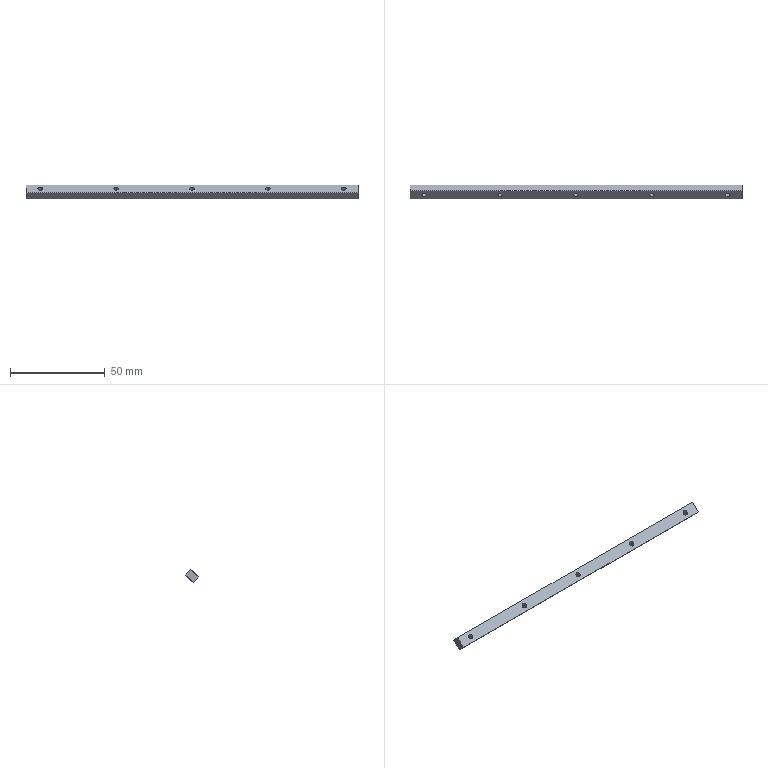Component | SolidWorks | FlatKey6-175-1 | 1 solid | 16 faces | box 175 x 7.31 x 7.25 mm | volume 4409 mm3 | cylinder 10 | plane 6 | commonest cylinder face diameters 2.5 x10 | material Alternative Material
build123d program:
from build123d import *

# Parameters (mm, degrees)
SKETCH1_W           = 175
SKETCH1_H           = 6
BOSS_EXTRUDE1_DEPTH = 4.3
M3_TAPPED_HOLE1_D   = 2.5


with BuildPart() as part:
    # Sketch1 → Boss-Extrude1 (new body)
    with BuildSketch(Plane.XY):
        Rectangle(SKETCH1_W, SKETCH1_H)
    extrude(amount=BOSS_EXTRUDE1_DEPTH)

    # M3 Tapped Hole1 (through all)
    with Locations(Plane.XY.offset(4.3)):
        with Locations((-80, 0), (-40, 0), (0, 0), (40, 0), (80, 0)):
            Hole(M3_TAPPED_HOLE1_D / 2)


solid = part.part

# Placed as in the assembly
solid = solid.moved(Location((-53.09, -33.192, -12.39), (43.57, 0, 0)))
STEP:
#1=COLOUR_RGB('',0.7922,0.8196,0.9333);
#2=FILL_AREA_STYLE_COLOUR('',#1);
#3=FILL_AREA_STYLE('',(#2));
#4=SURFACE_STYLE_FILL_AREA(#3);
#5=SURFACE_SIDE_STYLE('',(#4));
#6=SURFACE_STYLE_USAGE(.BOTH.,#5);
#7=PRESENTATION_STYLE_ASSIGNMENT((#6));
#8=CARTESIAN_POINT('',(-5.289,-1.423,-0.3652));
#9=VERTEX_POINT('',#8);
#10=CARTESIAN_POINT('',(-5.191,-1.423,-0.3652));
#11=VERTEX_POINT('',#10);
#12=CARTESIAN_POINT('',(-5.24,-1.423,-0.3652));
#13=DIRECTION('',(0.,0.6892,-0.7245));
#14=DIRECTION('',(1.,0.,0.));
#15=AXIS2_PLACEMENT_3D('',#12,#13,#14);
#16=CIRCLE('',#15,0.04921);
#17=EDGE_CURVE('',#9,#11,#16,.T.);
#18=ORIENTED_EDGE('',*,*,#17,.F.);
#19=CARTESIAN_POINT('',(-5.289,-1.307,-0.4878));
#20=VERTEX_POINT('',#19);
#21=CARTESIAN_POINT('',(-5.289,-1.307,-0.4878));
#22=DIRECTION('',(0.,0.6892,-0.7245));
#23=VECTOR('',#22,39.37);
#24=LINE('',#21,#23);
#25=EDGE_CURVE('',#9,#20,#24,.T.);
#26=ORIENTED_EDGE('',*,*,#25,.T.);
#27=CARTESIAN_POINT('',(-5.191,-1.307,-0.4878));
#28=VERTEX_POINT('',#27);
#29=CARTESIAN_POINT('',(-5.24,-1.307,-0.4878));
#30=DIRECTION('',(0.,0.6892,-0.7245));
#31=DIRECTION('',(1.,0.,0.));
#32=AXIS2_PLACEMENT_3D('',#29,#30,#31);
#33=CIRCLE('',#32,0.04921);
#34=EDGE_CURVE('',#20,#28,#33,.T.);
#35=ORIENTED_EDGE('',*,*,#34,.T.);
#36=CARTESIAN_POINT('',(-5.191,-1.307,-0.4878));
#37=DIRECTION('',(0.,0.6892,-0.7245));
#38=VECTOR('',#37,39.37);
#39=LINE('',#36,#38);
#40=EDGE_CURVE('',#11,#28,#39,.T.);
#41=ORIENTED_EDGE('',*,*,#40,.F.);
#42=EDGE_LOOP('',(#18,#26,#35,#41));
#43=FACE_OUTER_BOUND('',#42,.T.);
#44=CARTESIAN_POINT('',(-5.24,-1.307,-0.4878));
#45=DIRECTION('',(0.,0.6892,-0.7245));
#46=DIRECTION('',(1.,0.,0.));
#47=AXIS2_PLACEMENT_3D('',#44,#45,#46);
#48=CYLINDRICAL_SURFACE('',#47,0.04921);
#49=ADVANCED_FACE('',(#43),#48,.F.);
#50=CARTESIAN_POINT('',(-3.714,-1.423,-0.3652));
#51=VERTEX_POINT('',#50);
#52=CARTESIAN_POINT('',(-3.616,-1.423,-0.3652));
#53=VERTEX_POINT('',#52);
#54=CARTESIAN_POINT('',(-3.665,-1.423,-0.3652));
#55=DIRECTION('',(0.,0.6892,-0.7245));
#56=DIRECTION('',(1.,0.,0.));
#57=AXIS2_PLACEMENT_3D('',#54,#55,#56);
#58=CIRCLE('',#57,0.04921);
#59=EDGE_CURVE('',#51,#53,#58,.T.);
#60=ORIENTED_EDGE('',*,*,#59,.F.);
#61=CARTESIAN_POINT('',(-3.714,-1.307,-0.4878));
#62=VERTEX_POINT('',#61);
#63=CARTESIAN_POINT('',(-3.714,-1.307,-0.4878));
#64=DIRECTION('',(0.,0.6892,-0.7245));
#65=VECTOR('',#64,39.37);
#66=LINE('',#63,#65);
#67=EDGE_CURVE('',#51,#62,#66,.T.);
#68=ORIENTED_EDGE('',*,*,#67,.T.);
#69=CARTESIAN_POINT('',(-3.616,-1.307,-0.4878));
#70=VERTEX_POINT('',#69);
#71=CARTESIAN_POINT('',(-3.665,-1.307,-0.4878));
#72=DIRECTION('',(0.,0.6892,-0.7245));
#73=DIRECTION('',(1.,0.,0.));
#74=AXIS2_PLACEMENT_3D('',#71,#72,#73);
#75=CIRCLE('',#74,0.04921);
#76=EDGE_CURVE('',#62,#70,#75,.T.);
#77=ORIENTED_EDGE('',*,*,#76,.T.);
#78=CARTESIAN_POINT('',(-3.616,-1.307,-0.4878));
#79=DIRECTION('',(0.,0.6892,-0.7245));
#80=VECTOR('',#79,39.37);
#81=LINE('',#78,#80);
#82=EDGE_CURVE('',#53,#70,#81,.T.);
#83=ORIENTED_EDGE('',*,*,#82,.F.);
#84=EDGE_LOOP('',(#60,#68,#77,#83));
#85=FACE_OUTER_BOUND('',#84,.T.);
#86=CARTESIAN_POINT('',(-3.665,-1.307,-0.4878));
#87=DIRECTION('',(0.,0.6892,-0.7245));
#88=DIRECTION('',(1.,0.,0.));
#89=AXIS2_PLACEMENT_3D('',#86,#87,#88);
#90=CYLINDRICAL_SURFACE('',#89,0.04921);
#91=ADVANCED_FACE('',(#85),#90,.F.);
#92=CARTESIAN_POINT('',(-2.139,-1.423,-0.3652));
#93=VERTEX_POINT('',#92);
#94=CARTESIAN_POINT('',(-2.041,-1.423,-0.3652));
#95=VERTEX_POINT('',#94);
#96=CARTESIAN_POINT('',(-2.09,-1.423,-0.3652));
#97=DIRECTION('',(0.,0.6892,-0.7245));
#98=DIRECTION('',(1.,0.,0.));
#99=AXIS2_PLACEMENT_3D('',#96,#97,#98);
#100=CIRCLE('',#99,0.04921);
#101=EDGE_CURVE('',#93,#95,#100,.T.);
#102=ORIENTED_EDGE('',*,*,#101,.F.);
#103=CARTESIAN_POINT('',(-2.139,-1.307,-0.4878));
#104=VERTEX_POINT('',#103);
#105=CARTESIAN_POINT('',(-2.139,-1.307,-0.4878));
#106=DIRECTION('',(0.,0.6892,-0.7245));
#107=VECTOR('',#106,39.37);
#108=LINE('',#105,#107);
#109=EDGE_CURVE('',#93,#104,#108,.T.);
#110=ORIENTED_EDGE('',*,*,#109,.T.);
#111=CARTESIAN_POINT('',(-2.041,-1.307,-0.4878));
#112=VERTEX_POINT('',#111);
#113=CARTESIAN_POINT('',(-2.09,-1.307,-0.4878));
#114=DIRECTION('',(0.,0.6892,-0.7245));
#115=DIRECTION('',(1.,0.,0.));
#116=AXIS2_PLACEMENT_3D('',#113,#114,#115);
#117=CIRCLE('',#116,0.04921);
#118=EDGE_CURVE('',#104,#112,#117,.T.);
#119=ORIENTED_EDGE('',*,*,#118,.T.);
#120=CARTESIAN_POINT('',(-2.041,-1.307,-0.4878));
#121=DIRECTION('',(0.,0.6892,-0.7245));
#122=VECTOR('',#121,39.37);
#123=LINE('',#120,#122);
#124=EDGE_CURVE('',#95,#112,#123,.T.);
#125=ORIENTED_EDGE('',*,*,#124,.F.);
#126=EDGE_LOOP('',(#102,#110,#119,#125));
#127=FACE_OUTER_BOUND('',#126,.T.);
#128=CARTESIAN_POINT('',(-2.09,-1.307,-0.4878));
#129=DIRECTION('',(0.,0.6892,-0.7245));
#130=DIRECTION('',(1.,0.,0.));
#131=AXIS2_PLACEMENT_3D('',#128,#129,#130);
#132=CYLINDRICAL_SURFACE('',#131,0.04921);
#133=ADVANCED_FACE('',(#127),#132,.F.);
#134=CARTESIAN_POINT('',(-0.5646,-1.423,-0.3652));
#135=VERTEX_POINT('',#134);
#136=CARTESIAN_POINT('',(-0.4662,-1.423,-0.3652));
#137=VERTEX_POINT('',#136);
#138=CARTESIAN_POINT('',(-0.5154,-1.423,-0.3652));
#139=DIRECTION('',(0.,0.6892,-0.7245));
#140=DIRECTION('',(1.,0.,0.));
#141=AXIS2_PLACEMENT_3D('',#138,#139,#140);
#142=CIRCLE('',#141,0.04921);
#143=EDGE_CURVE('',#135,#137,#142,.T.);
#144=ORIENTED_EDGE('',*,*,#143,.F.);
#145=CARTESIAN_POINT('',(-0.5646,-1.307,-0.4878));
#146=VERTEX_POINT('',#145);
#147=CARTESIAN_POINT('',(-0.5646,-1.307,-0.4878));
#148=DIRECTION('',(0.,0.6892,-0.7245));
#149=VECTOR('',#148,39.37);
#150=LINE('',#147,#149);
#151=EDGE_CURVE('',#135,#146,#150,.T.);
#152=ORIENTED_EDGE('',*,*,#151,.T.);
#153=CARTESIAN_POINT('',(-0.4662,-1.307,-0.4878));
#154=VERTEX_POINT('',#153);
#155=CARTESIAN_POINT('',(-0.5154,-1.307,-0.4878));
#156=DIRECTION('',(0.,0.6892,-0.7245));
#157=DIRECTION('',(1.,0.,0.));
#158=AXIS2_PLACEMENT_3D('',#155,#156,#157);
#159=CIRCLE('',#158,0.04921);
#160=EDGE_CURVE('',#146,#154,#159,.T.);
#161=ORIENTED_EDGE('',*,*,#160,.T.);
#162=CARTESIAN_POINT('',(-0.4662,-1.307,-0.4878));
#163=DIRECTION('',(0.,0.6892,-0.7245));
#164=VECTOR('',#163,39.37);
#165=LINE('',#162,#164);
#166=EDGE_CURVE('',#137,#154,#165,.T.);
#167=ORIENTED_EDGE('',*,*,#166,.F.);
#168=EDGE_LOOP('',(#144,#152,#161,#167));
#169=FACE_OUTER_BOUND('',#168,.T.);
#170=CARTESIAN_POINT('',(-0.5154,-1.307,-0.4878));
#171=DIRECTION('',(0.,0.6892,-0.7245));
#172=DIRECTION('',(1.,0.,0.));
#173=AXIS2_PLACEMENT_3D('',#170,#171,#172);
#174=CYLINDRICAL_SURFACE('',#173,0.04921);
#175=ADVANCED_FACE('',(#169),#174,.F.);
#176=CARTESIAN_POINT('',(1.01,-1.423,-0.3652));
#177=VERTEX_POINT('',#176);
#178=CARTESIAN_POINT('',(1.109,-1.423,-0.3652));
#179=VERTEX_POINT('',#178);
#180=CARTESIAN_POINT('',(1.059,-1.423,-0.3652));
#181=DIRECTION('',(0.,0.6892,-0.7245));
#182=DIRECTION('',(1.,0.,0.));
#183=AXIS2_PLACEMENT_3D('',#180,#181,#182);
#184=CIRCLE('',#183,0.04921);
#185=EDGE_CURVE('',#177,#179,#184,.T.);
#186=ORIENTED_EDGE('',*,*,#185,.F.);
#187=CARTESIAN_POINT('',(1.01,-1.307,-0.4878));
#188=VERTEX_POINT('',#187);
#189=CARTESIAN_POINT('',(1.01,-1.307,-0.4878));
#190=DIRECTION('',(0.,0.6892,-0.7245));
#191=VECTOR('',#190,39.37);
#192=LINE('',#189,#191);
#193=EDGE_CURVE('',#177,#188,#192,.T.);
#194=ORIENTED_EDGE('',*,*,#193,.T.);
#195=CARTESIAN_POINT('',(1.109,-1.307,-0.4878));
#196=VERTEX_POINT('',#195);
#197=CARTESIAN_POINT('',(1.059,-1.307,-0.4878));
#198=DIRECTION('',(0.,0.6892,-0.7245));
#199=DIRECTION('',(1.,0.,0.));
#200=AXIS2_PLACEMENT_3D('',#197,#198,#199);
#201=CIRCLE('',#200,0.04921);
#202=EDGE_CURVE('',#188,#196,#201,.T.);
#203=ORIENTED_EDGE('',*,*,#202,.T.);
#204=CARTESIAN_POINT('',(1.109,-1.307,-0.4878));
#205=DIRECTION('',(0.,0.6892,-0.7245));
#206=VECTOR('',#205,39.37);
#207=LINE('',#204,#206);
#208=EDGE_CURVE('',#179,#196,#207,.T.);
#209=ORIENTED_EDGE('',*,*,#208,.F.);
#210=EDGE_LOOP('',(#186,#194,#203,#209));
#211=FACE_OUTER_BOUND('',#210,.T.);
#212=CARTESIAN_POINT('',(1.059,-1.307,-0.4878));
#213=DIRECTION('',(0.,0.6892,-0.7245));
#214=DIRECTION('',(1.,0.,0.));
#215=AXIS2_PLACEMENT_3D('',#212,#213,#214);
#216=CYLINDRICAL_SURFACE('',#215,0.04921);
#217=ADVANCED_FACE('',(#211),#216,.F.);
#218=CARTESIAN_POINT('',(1.355,-1.338,-0.2837));
#219=VERTEX_POINT('',#218);
#220=CARTESIAN_POINT('',(1.355,-1.509,-0.4466));
#221=VERTEX_POINT('',#220);
#222=CARTESIAN_POINT('',(1.355,-1.338,-0.2837));
#223=DIRECTION('',(0.,-0.7245,-0.6892));
#224=VECTOR('',#223,39.37);
#225=LINE('',#222,#224);
#226=EDGE_CURVE('',#219,#221,#225,.T.);
#227=ORIENTED_EDGE('',*,*,#226,.T.);
#228=CARTESIAN_POINT('',(1.355,-1.392,-0.5692));
#229=VERTEX_POINT('',#228);
#230=CARTESIAN_POINT('',(1.355,-1.392,-0.5692));
#231=DIRECTION('',(0.,-0.6892,0.7245));
#232=VECTOR('',#231,39.37);
#233=LINE('',#230,#232);
#234=EDGE_CURVE('',#229,#221,#233,.T.);
#235=ORIENTED_EDGE('',*,*,#234,.F.);
#236=CARTESIAN_POINT('',(1.355,-1.221,-0.4064));
#237=VERTEX_POINT('',#236);
#238=CARTESIAN_POINT('',(1.355,-1.221,-0.4064));
#239=DIRECTION('',(0.,-0.7245,-0.6892));
#240=VECTOR('',#239,39.37);
#241=LINE('',#238,#240);
#242=EDGE_CURVE('',#237,#229,#241,.T.);
#243=ORIENTED_EDGE('',*,*,#242,.F.);
#244=CARTESIAN_POINT('',(1.355,-1.221,-0.4064));
#245=DIRECTION('',(0.,-0.6892,0.7245));
#246=VECTOR('',#245,39.37);
#247=LINE('',#244,#246);
#248=EDGE_CURVE('',#237,#219,#247,.T.);
#249=ORIENTED_EDGE('',*,*,#248,.T.);
#250=EDGE_LOOP('',(#227,#235,#243,#249));
#251=FACE_OUTER_BOUND('',#250,.T.);
#252=CARTESIAN_POINT('',(1.355,-1.221,-0.4064));
#253=DIRECTION('',(-1.,0.,0.));
#254=DIRECTION('',(0.,0.6892,-0.7245));
#255=AXIS2_PLACEMENT_3D('',#252,#253,#254);
#256=PLANE('',#255);
#257=ADVANCED_FACE('',(#251),#256,.F.);
#258=CARTESIAN_POINT('',(-5.535,-1.509,-0.4466));
#259=VERTEX_POINT('',#258);
#260=CARTESIAN_POINT('',(-5.535,-1.509,-0.4466));
#261=DIRECTION('',(-1.,0.,0.));
#262=VECTOR('',#261,39.37);
#263=LINE('',#260,#262);
#264=EDGE_CURVE('',#221,#259,#263,.T.);
#265=ORIENTED_EDGE('',*,*,#264,.T.);
#266=CARTESIAN_POINT('',(-5.535,-1.392,-0.5692));
#267=VERTEX_POINT('',#266);
#268=CARTESIAN_POINT('',(-5.535,-1.392,-0.5692));
#269=DIRECTION('',(0.,-0.6892,0.7245));
#270=VECTOR('',#269,39.37);
#271=LINE('',#268,#270);
#272=EDGE_CURVE('',#267,#259,#271,.T.);
#273=ORIENTED_EDGE('',*,*,#272,.F.);
#274=CARTESIAN_POINT('',(-5.535,-1.392,-0.5692));
#275=DIRECTION('',(-1.,0.,0.));
#276=VECTOR('',#275,39.37);
#277=LINE('',#274,#276);
#278=EDGE_CURVE('',#229,#267,#277,.T.);
#279=ORIENTED_EDGE('',*,*,#278,.F.);
#280=ORIENTED_EDGE('',*,*,#234,.T.);
#281=EDGE_LOOP('',(#265,#273,#279,#280));
#282=FACE_OUTER_BOUND('',#281,.T.);
#283=CARTESIAN_POINT('',(-5.535,-1.392,-0.5692));
#284=DIRECTION('',(0.,0.7245,0.6892));
#285=DIRECTION('',(0.,-0.6892,0.7245));
#286=AXIS2_PLACEMENT_3D('',#283,#284,#285);
#287=PLANE('',#286);
#288=ADVANCED_FACE('',(#282),#287,.F.);
#289=CARTESIAN_POINT('',(-5.535,-1.338,-0.2837));
#290=VERTEX_POINT('',#289);
#291=CARTESIAN_POINT('',(-5.535,-1.338,-0.2837));
#292=DIRECTION('',(0.,0.7245,0.6892));
#293=VECTOR('',#292,39.37);
#294=LINE('',#291,#293);
#295=EDGE_CURVE('',#259,#290,#294,.T.);
#296=ORIENTED_EDGE('',*,*,#295,.T.);
#297=CARTESIAN_POINT('',(-5.535,-1.221,-0.4064));
#298=VERTEX_POINT('',#297);
#299=CARTESIAN_POINT('',(-5.535,-1.221,-0.4064));
#300=DIRECTION('',(0.,-0.6892,0.7245));
#301=VECTOR('',#300,39.37);
#302=LINE('',#299,#301);
#303=EDGE_CURVE('',#298,#290,#302,.T.);
#304=ORIENTED_EDGE('',*,*,#303,.F.);
#305=CARTESIAN_POINT('',(-5.535,-1.221,-0.4064));
#306=DIRECTION('',(0.,0.7245,0.6892));
#307=VECTOR('',#306,39.37);
#308=LINE('',#305,#307);
#309=EDGE_CURVE('',#267,#298,#308,.T.);
#310=ORIENTED_EDGE('',*,*,#309,.F.);
#311=ORIENTED_EDGE('',*,*,#272,.T.);
#312=EDGE_LOOP('',(#296,#304,#310,#311));
#313=FACE_OUTER_BOUND('',#312,.T.);
#314=CARTESIAN_POINT('',(-5.535,-1.221,-0.4064));
#315=DIRECTION('',(1.,0.,0.));
#316=DIRECTION('',(0.,-0.6892,0.7245));
#317=AXIS2_PLACEMENT_3D('',#314,#315,#316);
#318=PLANE('',#317);
#319=ADVANCED_FACE('',(#313),#318,.F.);
#320=CARTESIAN_POINT('',(-5.535,-1.338,-0.2837));
#321=DIRECTION('',(1.,0.,0.));
#322=VECTOR('',#321,39.37);
#323=LINE('',#320,#322);
#324=EDGE_CURVE('',#290,#219,#323,.T.);
#325=ORIENTED_EDGE('',*,*,#324,.T.);
#326=ORIENTED_EDGE('',*,*,#248,.F.);
#327=CARTESIAN_POINT('',(-5.535,-1.221,-0.4064));
#328=DIRECTION('',(1.,0.,0.));
#329=VECTOR('',#328,39.37);
#330=LINE('',#327,#329);
#331=EDGE_CURVE('',#298,#237,#330,.T.);
#332=ORIENTED_EDGE('',*,*,#331,.F.);
#333=ORIENTED_EDGE('',*,*,#303,.T.);
#334=EDGE_LOOP('',(#325,#326,#332,#333));
#335=FACE_OUTER_BOUND('',#334,.T.);
#336=CARTESIAN_POINT('',(-5.535,-1.221,-0.4064));
#337=DIRECTION('',(0.,-0.7245,-0.6892));
#338=DIRECTION('',(0.,0.6892,-0.7245));
#339=AXIS2_PLACEMENT_3D('',#336,#337,#338);
#340=PLANE('',#339);
#341=ADVANCED_FACE('',(#335),#340,.F.);
#342=CARTESIAN_POINT('',(-5.24,-1.307,-0.4878));
#343=DIRECTION('',(0.,0.6892,-0.7245));
#344=DIRECTION('',(1.,0.,0.));
#345=AXIS2_PLACEMENT_3D('',#342,#343,#344);
#346=CIRCLE('',#345,0.04921);
#347=EDGE_CURVE('',#28,#20,#346,.T.);
#348=ORIENTED_EDGE('',*,*,#347,.F.);
#349=ORIENTED_EDGE('',*,*,#34,.F.);
#350=EDGE_LOOP('',(#348,#349));
#351=FACE_BOUND('',#350,.T.);
#352=CARTESIAN_POINT('',(-3.665,-1.307,-0.4878));
#353=DIRECTION('',(0.,0.6892,-0.7245));
#354=DIRECTION('',(1.,0.,0.));
#355=AXIS2_PLACEMENT_3D('',#352,#353,#354);
#356=CIRCLE('',#355,0.04921);
#357=EDGE_CURVE('',#70,#62,#356,.T.);
#358=ORIENTED_EDGE('',*,*,#357,.F.);
#359=ORIENTED_EDGE('',*,*,#76,.F.);
#360=EDGE_LOOP('',(#358,#359));
#361=FACE_BOUND('',#360,.T.);
#362=CARTESIAN_POINT('',(-2.09,-1.307,-0.4878));
#363=DIRECTION('',(0.,0.6892,-0.7245));
#364=DIRECTION('',(1.,0.,0.));
#365=AXIS2_PLACEMENT_3D('',#362,#363,#364);
#366=CIRCLE('',#365,0.04921);
#367=EDGE_CURVE('',#112,#104,#366,.T.);
#368=ORIENTED_EDGE('',*,*,#367,.F.);
#369=ORIENTED_EDGE('',*,*,#118,.F.);
#370=EDGE_LOOP('',(#368,#369));
#371=FACE_BOUND('',#370,.T.);
#372=CARTESIAN_POINT('',(-0.5154,-1.307,-0.4878));
#373=DIRECTION('',(0.,0.6892,-0.7245));
#374=DIRECTION('',(1.,0.,0.));
#375=AXIS2_PLACEMENT_3D('',#372,#373,#374);
#376=CIRCLE('',#375,0.04921);
#377=EDGE_CURVE('',#154,#146,#376,.T.);
#378=ORIENTED_EDGE('',*,*,#377,.F.);
#379=ORIENTED_EDGE('',*,*,#160,.F.);
#380=EDGE_LOOP('',(#378,#379));
#381=FACE_BOUND('',#380,.T.);
#382=CARTESIAN_POINT('',(1.059,-1.307,-0.4878));
#383=DIRECTION('',(0.,0.6892,-0.7245));
#384=DIRECTION('',(1.,0.,0.));
#385=AXIS2_PLACEMENT_3D('',#382,#383,#384);
#386=CIRCLE('',#385,0.04921);
#387=EDGE_CURVE('',#196,#188,#386,.T.);
#388=ORIENTED_EDGE('',*,*,#387,.F.);
#389=ORIENTED_EDGE('',*,*,#202,.F.);
#390=EDGE_LOOP('',(#388,#389));
#391=FACE_BOUND('',#390,.T.);
#392=ORIENTED_EDGE('',*,*,#242,.T.);
#393=ORIENTED_EDGE('',*,*,#278,.T.);
#394=ORIENTED_EDGE('',*,*,#309,.T.);
#395=ORIENTED_EDGE('',*,*,#331,.T.);
#396=EDGE_LOOP('',(#392,#393,#394,#395));
#397=FACE_OUTER_BOUND('',#396,.T.);
#398=CARTESIAN_POINT('',(1.355,-1.392,-0.5692));
#399=DIRECTION('',(0.,-0.6892,0.7245));
#400=DIRECTION('',(-1.,0.,0.));
#401=AXIS2_PLACEMENT_3D('',#398,#399,#400);
#402=PLANE('',#401);
#403=ADVANCED_FACE('',(#351,#361,#371,#381,#391,#397),#402,.F.);
#404=CARTESIAN_POINT('',(-5.24,-1.423,-0.3652));
#405=DIRECTION('',(0.,0.6892,-0.7245));
#406=DIRECTION('',(1.,0.,0.));
#407=AXIS2_PLACEMENT_3D('',#404,#405,#406);
#408=CIRCLE('',#407,0.04921);
#409=EDGE_CURVE('',#11,#9,#408,.T.);
#410=ORIENTED_EDGE('',*,*,#409,.T.);
#411=ORIENTED_EDGE('',*,*,#17,.T.);
#412=EDGE_LOOP('',(#410,#411));
#413=FACE_BOUND('',#412,.T.);
#414=CARTESIAN_POINT('',(-3.665,-1.423,-0.3652));
#415=DIRECTION('',(0.,0.6892,-0.7245));
#416=DIRECTION('',(1.,0.,0.));
#417=AXIS2_PLACEMENT_3D('',#414,#415,#416);
#418=CIRCLE('',#417,0.04921);
#419=EDGE_CURVE('',#53,#51,#418,.T.);
#420=ORIENTED_EDGE('',*,*,#419,.T.);
#421=ORIENTED_EDGE('',*,*,#59,.T.);
#422=EDGE_LOOP('',(#420,#421));
#423=FACE_BOUND('',#422,.T.);
#424=CARTESIAN_POINT('',(-2.09,-1.423,-0.3652));
#425=DIRECTION('',(0.,0.6892,-0.7245));
#426=DIRECTION('',(1.,0.,0.));
#427=AXIS2_PLACEMENT_3D('',#424,#425,#426);
#428=CIRCLE('',#427,0.04921);
#429=EDGE_CURVE('',#95,#93,#428,.T.);
#430=ORIENTED_EDGE('',*,*,#429,.T.);
#431=ORIENTED_EDGE('',*,*,#101,.T.);
#432=EDGE_LOOP('',(#430,#431));
#433=FACE_BOUND('',#432,.T.);
#434=CARTESIAN_POINT('',(-0.5154,-1.423,-0.3652));
#435=DIRECTION('',(0.,0.6892,-0.7245));
#436=DIRECTION('',(1.,0.,0.));
#437=AXIS2_PLACEMENT_3D('',#434,#435,#436);
#438=CIRCLE('',#437,0.04921);
#439=EDGE_CURVE('',#137,#135,#438,.T.);
#440=ORIENTED_EDGE('',*,*,#439,.T.);
#441=ORIENTED_EDGE('',*,*,#143,.T.);
#442=EDGE_LOOP('',(#440,#441));
#443=FACE_BOUND('',#442,.T.);
#444=CARTESIAN_POINT('',(1.059,-1.423,-0.3652));
#445=DIRECTION('',(0.,0.6892,-0.7245));
#446=DIRECTION('',(1.,0.,0.));
#447=AXIS2_PLACEMENT_3D('',#444,#445,#446);
#448=CIRCLE('',#447,0.04921);
#449=EDGE_CURVE('',#179,#177,#448,.T.);
#450=ORIENTED_EDGE('',*,*,#449,.T.);
#451=ORIENTED_EDGE('',*,*,#185,.T.);
#452=EDGE_LOOP('',(#450,#451));
#453=FACE_BOUND('',#452,.T.);
#454=ORIENTED_EDGE('',*,*,#226,.F.);
#455=ORIENTED_EDGE('',*,*,#324,.F.);
#456=ORIENTED_EDGE('',*,*,#295,.F.);
#457=ORIENTED_EDGE('',*,*,#264,.F.);
#458=EDGE_LOOP('',(#454,#455,#456,#457));
#459=FACE_OUTER_BOUND('',#458,.T.);
#460=CARTESIAN_POINT('',(1.355,-1.509,-0.4466));
#461=DIRECTION('',(0.,-0.6892,0.7245));
#462=DIRECTION('',(-1.,0.,0.));
#463=AXIS2_PLACEMENT_3D('',#460,#461,#462);
#464=PLANE('',#463);
#465=ADVANCED_FACE('',(#413,#423,#433,#443,#453,#459),#464,.T.);
#466=ORIENTED_EDGE('',*,*,#193,.F.);
#467=ORIENTED_EDGE('',*,*,#449,.F.);
#468=ORIENTED_EDGE('',*,*,#208,.T.);
#469=ORIENTED_EDGE('',*,*,#387,.T.);
#470=EDGE_LOOP('',(#466,#467,#468,#469));
#471=FACE_OUTER_BOUND('',#470,.T.);
#472=CARTESIAN_POINT('',(1.059,-1.307,-0.4878));
#473=DIRECTION('',(0.,0.6892,-0.7245));
#474=DIRECTION('',(1.,0.,0.));
#475=AXIS2_PLACEMENT_3D('',#472,#473,#474);
#476=CYLINDRICAL_SURFACE('',#475,0.04921);
#477=ADVANCED_FACE('',(#471),#476,.F.);
#478=ORIENTED_EDGE('',*,*,#151,.F.);
#479=ORIENTED_EDGE('',*,*,#439,.F.);
#480=ORIENTED_EDGE('',*,*,#166,.T.);
#481=ORIENTED_EDGE('',*,*,#377,.T.);
#482=EDGE_LOOP('',(#478,#479,#480,#481));
#483=FACE_OUTER_BOUND('',#482,.T.);
#484=CARTESIAN_POINT('',(-0.5154,-1.307,-0.4878));
#485=DIRECTION('',(0.,0.6892,-0.7245));
#486=DIRECTION('',(1.,0.,0.));
#487=AXIS2_PLACEMENT_3D('',#484,#485,#486);
#488=CYLINDRICAL_SURFACE('',#487,0.04921);
#489=ADVANCED_FACE('',(#483),#488,.F.);
#490=ORIENTED_EDGE('',*,*,#109,.F.);
#491=ORIENTED_EDGE('',*,*,#429,.F.);
#492=ORIENTED_EDGE('',*,*,#124,.T.);
#493=ORIENTED_EDGE('',*,*,#367,.T.);
#494=EDGE_LOOP('',(#490,#491,#492,#493));
#495=FACE_OUTER_BOUND('',#494,.T.);
#496=CARTESIAN_POINT('',(-2.09,-1.307,-0.4878));
#497=DIRECTION('',(0.,0.6892,-0.7245));
#498=DIRECTION('',(1.,0.,0.));
#499=AXIS2_PLACEMENT_3D('',#496,#497,#498);
#500=CYLINDRICAL_SURFACE('',#499,0.04921);
#501=ADVANCED_FACE('',(#495),#500,.F.);
#502=ORIENTED_EDGE('',*,*,#67,.F.);
#503=ORIENTED_EDGE('',*,*,#419,.F.);
#504=ORIENTED_EDGE('',*,*,#82,.T.);
#505=ORIENTED_EDGE('',*,*,#357,.T.);
#506=EDGE_LOOP('',(#502,#503,#504,#505));
#507=FACE_OUTER_BOUND('',#506,.T.);
#508=CARTESIAN_POINT('',(-3.665,-1.307,-0.4878));
#509=DIRECTION('',(0.,0.6892,-0.7245));
#510=DIRECTION('',(1.,0.,0.));
#511=AXIS2_PLACEMENT_3D('',#508,#509,#510);
#512=CYLINDRICAL_SURFACE('',#511,0.04921);
#513=ADVANCED_FACE('',(#507),#512,.F.);
#514=ORIENTED_EDGE('',*,*,#25,.F.);
#515=ORIENTED_EDGE('',*,*,#409,.F.);
#516=ORIENTED_EDGE('',*,*,#40,.T.);
#517=ORIENTED_EDGE('',*,*,#347,.T.);
#518=EDGE_LOOP('',(#514,#515,#516,#517));
#519=FACE_OUTER_BOUND('',#518,.T.);
#520=CARTESIAN_POINT('',(-5.24,-1.307,-0.4878));
#521=DIRECTION('',(0.,0.6892,-0.7245));
#522=DIRECTION('',(1.,0.,0.));
#523=AXIS2_PLACEMENT_3D('',#520,#521,#522);
#524=CYLINDRICAL_SURFACE('',#523,0.04921);
#525=ADVANCED_FACE('',(#519),#524,.F.);
#526=CLOSED_SHELL('',(#49,#91,#133,#175,#217,#257,#288,#319,#341,#403,#465,#477,#489,#501,#513,#525));
#527=MANIFOLD_SOLID_BREP('',#526);
#528=STYLED_ITEM('',(#7),#527);
#529=PRESENTATION_LAYER_ASSIGNMENT('','',(#528));
#530=CARTESIAN_POINT('',(0.,0.,0.));
#531=DIRECTION('',(0.,0.,1.));
#532=DIRECTION('',(1.,0.,0.));
#533=AXIS2_PLACEMENT_3D('',#530,#531,#532);
#534=(LENGTH_UNIT()NAMED_UNIT(*)SI_UNIT($,.METRE.));
#535=LENGTH_MEASURE_WITH_UNIT(LENGTH_MEASURE(0.0254),#534);
#536=DIMENSIONAL_EXPONENTS(1.,0.,0.,0.,0.,0.,0.);
#537=(CONVERSION_BASED_UNIT('',#535)LENGTH_UNIT()NAMED_UNIT(#536));
#538=UNCERTAINTY_MEASURE_WITH_UNIT(LENGTH_MEASURE(0.00001),#537,'','');
#539=(NAMED_UNIT(*)PLANE_ANGLE_UNIT()SI_UNIT($,.RADIAN.));
#540=(NAMED_UNIT(*)SI_UNIT($,.STERADIAN.)SOLID_ANGLE_UNIT());
#541=(GEOMETRIC_REPRESENTATION_CONTEXT(3)GLOBAL_UNCERTAINTY_ASSIGNED_CONTEXT((#538))GLOBAL_UNIT_ASSIGNED_CONTEXT((#537,#539,#540))REPRESENTATION_CONTEXT('',''));
#542=ADVANCED_BREP_SHAPE_REPRESENTATION('',(#527,#533),#541);
#543=(LENGTH_UNIT()NAMED_UNIT(*)SI_UNIT($,.METRE.));
#544=LENGTH_MEASURE_WITH_UNIT(LENGTH_MEASURE(0.0254),#543);
#545=DIMENSIONAL_EXPONENTS(1.,0.,0.,0.,0.,0.,0.);
#546=(CONVERSION_BASED_UNIT('',#544)LENGTH_UNIT()NAMED_UNIT(#545));
#547=UNCERTAINTY_MEASURE_WITH_UNIT(LENGTH_MEASURE(0.00001),#546,'','');
#548=(NAMED_UNIT(*)PLANE_ANGLE_UNIT()SI_UNIT($,.RADIAN.));
#549=(NAMED_UNIT(*)SI_UNIT($,.STERADIAN.)SOLID_ANGLE_UNIT());
#550=(GEOMETRIC_REPRESENTATION_CONTEXT(3)GLOBAL_UNCERTAINTY_ASSIGNED_CONTEXT((#547))GLOBAL_UNIT_ASSIGNED_CONTEXT((#546,#548,#549))REPRESENTATION_CONTEXT('',''));
#551=MECHANICAL_DESIGN_GEOMETRIC_PRESENTATION_REPRESENTATION('',(#528),#550);